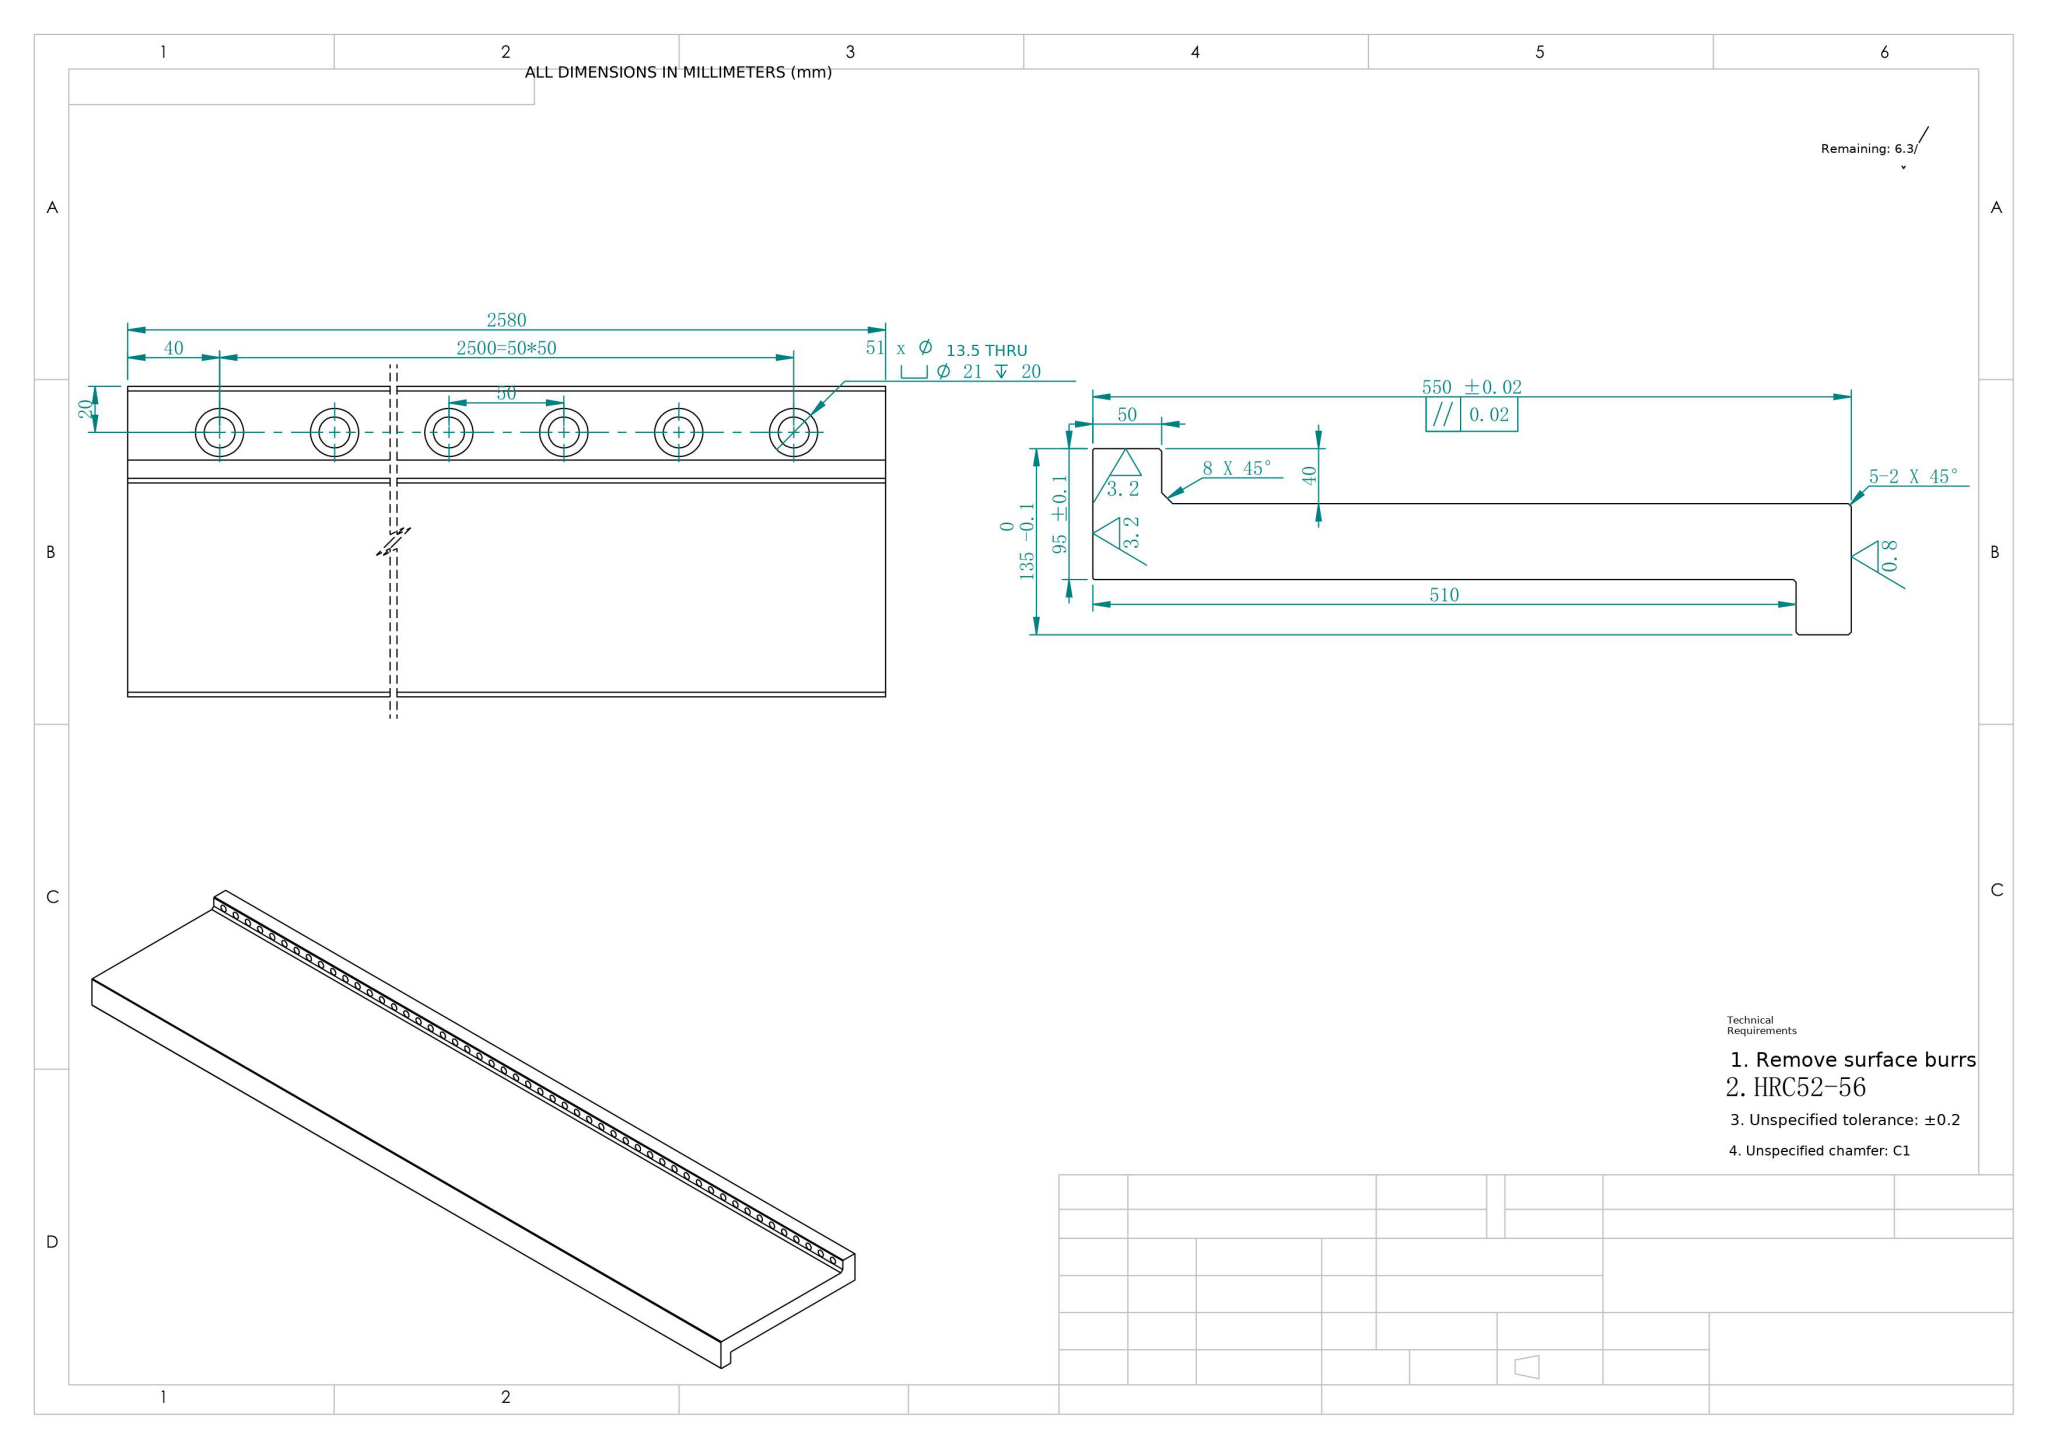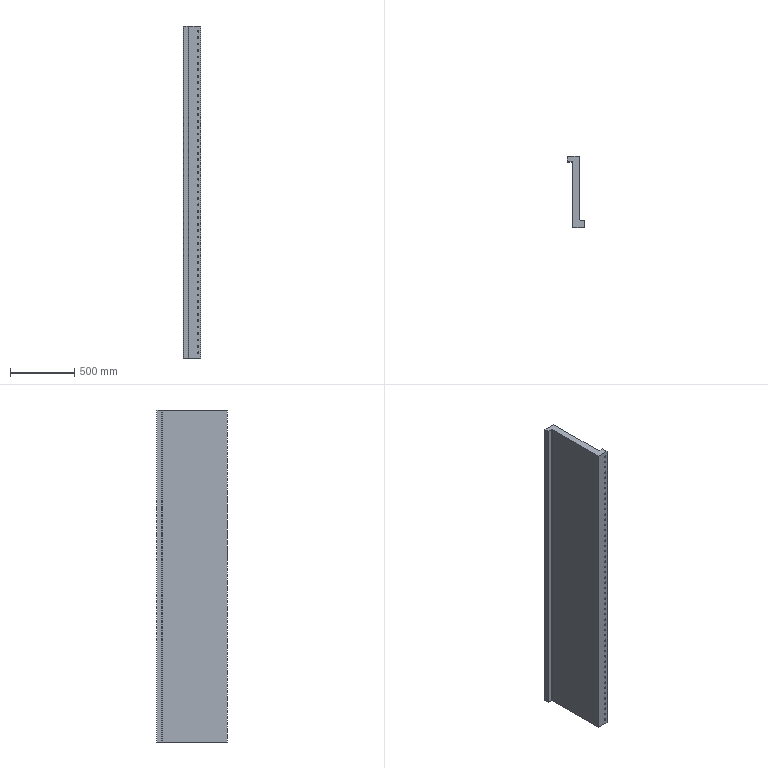Part | NX | mm | 1 solid | 273 faces | box 135 x 550 x 2580 mm | volume 86825210 mm3 | cylinder 204 | plane 69 | commonest cylinder face diameters 21 x102 13.5 x102